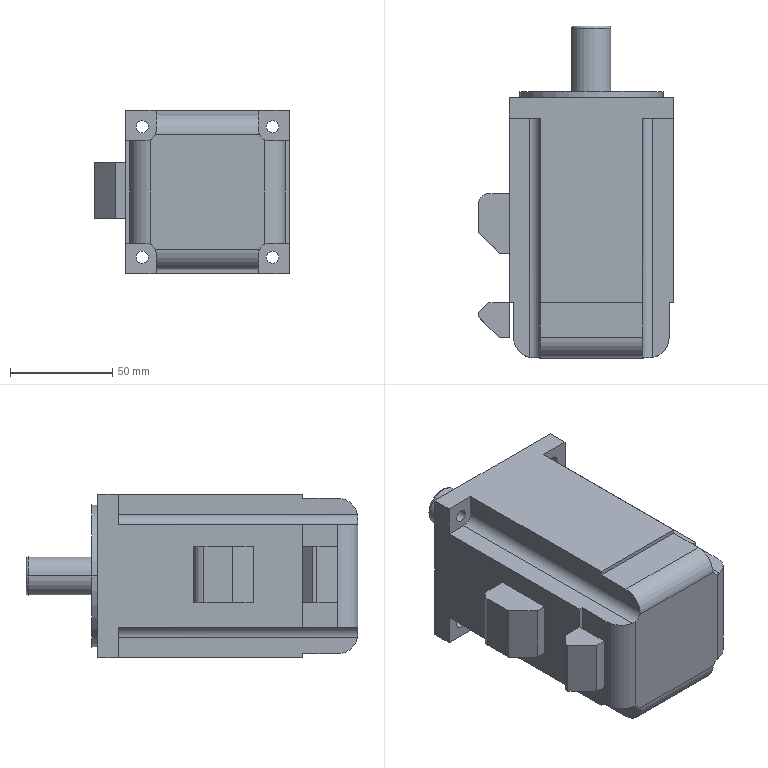Component | SolidWorks | 750WServoMotor(ML)A-1 | 2 solids | 68 faces | box 95 x 162 x 80 mm | volume 728960 mm3 | plane 43 | cylinder 23 | torus 2 | commonest cylinder face diameters 6 x8 10 x5 20 x4 19 x2 30 x2 70 x2
build123d program:
from build123d import *

# Parameters (mm, degrees)
SKETCH1_W            = 80
SKETCH1_H            = 80
BOSS_EXTRUDE1_DEPTH  = 100
SKETCH2_W            = 76
SKETCH2_H            = 76
BOSS_EXTRUDE2_DEPTH  = 27
FILLET1_R            = 10
SKETCH3_R            = 35
SKETCH3_R_2          = 15
BOSS_EXTRUDE3_DEPTH  = 3
SKETCH4_R            = 9.5
BOSS_EXTRUDE4_DEPTH  = 35
FILLET2_R            = 1
SKETCH5_W            = 17
SKETCH5_H            = 27.653
SKETCH5_W_2          = 29.036
BOSS_EXTRUDE5_DEPTH  = 15
CHAMFER1_SIZE        = 10
CHAMFER2_SIZE        = 10
FILLET3_R            = 5
CHAMFER3_SIZE        = 5
SKETCH6_R            = 3
CUT_EXTRUDE1_DEPTH   = 10
CUT_EXTRUDE2_DEPTH   = 136.329
MIRROR2_COPY_1_DEPTH = 136.329


with BuildPart() as part:
    # Sketch1 → Boss-Extrude1 (new body)
    with BuildSketch(Plane.XY):
        Rectangle(SKETCH1_W, SKETCH1_H)
    extrude(amount=BOSS_EXTRUDE1_DEPTH)

    # Sketch2 → Boss-Extrude2 (add)
    with BuildSketch(Plane.XY.offset(100)):
        Rectangle(SKETCH2_W, SKETCH2_H)
    extrude(amount=BOSS_EXTRUDE2_DEPTH)

    # Fillet1
    fillet1_edges = [part.edges().sort_by_distance(p)[0] for p in [
        (38, 0, 127),
        (0, 38, 127),
        (-38, 0, 127),
        (0, -38, 127),
    ]]
    fillet(fillet1_edges, radius=FILLET1_R)

    # Sketch3 → Boss-Extrude3 (add)
    with BuildSketch(Plane(origin=(0, 0, 0), x_dir=(-1, 0, 0), z_dir=(0, 0, -1))):
        with Locations(Location((0, 0, 0), (0, 0, 180))):
            Circle(SKETCH3_R)
        Circle(SKETCH3_R_2, mode=Mode.SUBTRACT)
    extrude(amount=BOSS_EXTRUDE3_DEPTH)

    # Sketch4 → Boss-Extrude4 (add)
    with BuildSketch(Plane(origin=(0, 0, 0), x_dir=(-1, 0, 0), z_dir=(0, 0, -1))):
        with Locations(Location((0, 0, 0), (0, 0, 180))):
            Circle(SKETCH4_R)
    extrude(amount=BOSS_EXTRUDE4_DEPTH)

    # Fillet2
    fillet2_edges = [part.edges().sort_by_distance(p)[0] for p in [
        (-9.5, 0, -35),
    ]]
    fillet(fillet2_edges, radius=FILLET2_R)

    # Sketch5 → Boss-Extrude5 (add)
    with BuildSketch(Plane.ZY.offset(40)):
        with Locations((108.5, 0.6913)):
            Rectangle(SKETCH5_W, SKETCH5_H)
        with Locations((61.348, 0.6913)):
            Rectangle(SKETCH5_W_2, SKETCH5_H)
    extrude(amount=BOSS_EXTRUDE5_DEPTH)


with BuildPart() as boss_extrude5_piece_1:
    # of the separate pieces the step leaves, piece 1, a body of its own (boss_extrude5_pieces)
    add(part.part.solids().sort_by_distance((9.5, 0, -34))[0])

    # Chamfer1
    chamfer1_edges = [boss_extrude5_piece_1.edges().sort_by_distance(p)[0] for p in [
        (-55, 0.6913, 75.866),
    ]]
    chamfer(chamfer1_edges, length=CHAMFER1_SIZE)

    # Fillet3
    fillet3_edges = [boss_extrude5_piece_1.edges().sort_by_distance(p)[0] for p in [
        (-55, 0.6913, 46.83),
    ]]
    fillet(fillet3_edges, radius=FILLET3_R)

    # Sketch6 → Cut-Extrude1 (cut)
    with BuildSketch(Plane(origin=(0, 0, 0), x_dir=(-1, 0, 0), z_dir=(0, 0, -1))):
        with Locations((-31.82, 31.82)):
            Circle(SKETCH6_R)
        with Locations(Location((-31.82, -31.82, 0), (0, 0, 180))):
            Circle(SKETCH6_R)
        with Locations((31.82, -31.82)):
            Circle(SKETCH6_R)
        with Locations(Location((31.82, 31.82, 0), (0, 0, 180))):
            Circle(SKETCH6_R)
    extrude(amount=-CUT_EXTRUDE1_DEPTH, mode=Mode.SUBTRACT)

    # Sketch7 → Cut-Extrude2 (cut, through all)
    with BuildSketch(Plane(origin=(0, 0, 10), x_dir=(-1, 0, 0), z_dir=(0, 0, -1))):
        with BuildLine():
            Line((-40, 40), (-25, 40))
            Line((-25, 40), (-25, 30))
            ThreePointArc((-25, 30), (-26.464, 26.464), (-30, 25))
            Line((-30, 25), (-40, 25))
            Line((-40, 25), (-40, 40))
        make_face()
    cut_extrude2 = extrude(amount=-CUT_EXTRUDE2_DEPTH, mode=Mode.SUBTRACT)

    # Mirror1: Cut-Extrude2 across plane
    add(cut_extrude2.mirror(Plane.ZX), mode=Mode.SUBTRACT)

    # Mirror2: Cut-Extrude2 across plane
    add(cut_extrude2.mirror(Plane(origin=(0, 0, 0), x_dir=(0, 0, 1), z_dir=(1, 0, 0))), mode=Mode.SUBTRACT)

    # Mirror2 copy 1 sketch → Mirror2 copy 1 (cut, through all)
    with BuildSketch(Plane(origin=(0, 0, 10), x_dir=(1, 0, 0), z_dir=(0, 0, -1))):
        with BuildLine():
            Line((-40, 40), (-25, 40))
            Line((-25, 40), (-25, 30))
            ThreePointArc((-25, 30), (-26.464, 26.464), (-30, 25))
            Line((-30, 25), (-40, 25))
            Line((-40, 25), (-40, 40))
        make_face()
    extrude(amount=-MIRROR2_COPY_1_DEPTH, mode=Mode.SUBTRACT)


with BuildPart() as boss_extrude5_piece_2:
    # of the separate pieces the step leaves, piece 2, a body of its own (boss_extrude5_pieces)
    add(part.part.solids().sort_by_distance((-55, 14.518, 100))[0])

    # Chamfer2
    chamfer2_edges = [boss_extrude5_piece_2.edges().sort_by_distance(p)[0] for p in [
        (-55, 0.6913, 117),
    ]]
    chamfer(chamfer2_edges, length=CHAMFER2_SIZE)

    # Chamfer3
    chamfer3_edges = [boss_extrude5_piece_2.edges().sort_by_distance(p)[0] for p in [
        (-55, 0.6913, 100),
    ]]
    chamfer(chamfer3_edges, length=CHAMFER3_SIZE)


solid = Compound([boss_extrude5_piece_1.part, boss_extrude5_piece_2.part])

# Placed as in the assembly
solid = solid.moved(Location((-864.885, -524.907, 1035.102), (90, 0, 0)))